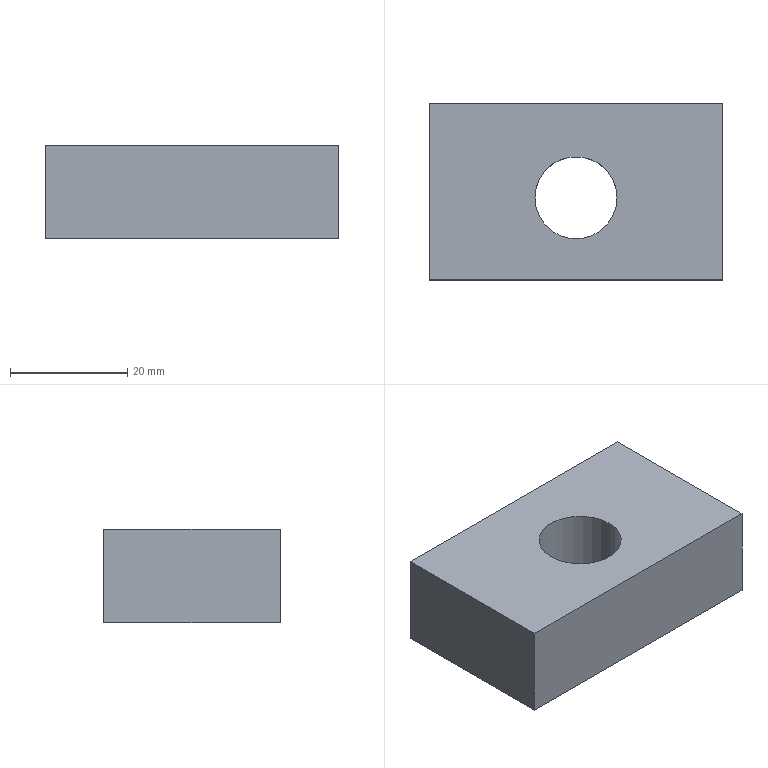Component | SolidWorks | TractionHandwheelAdjustmentPlate-1 | 1 solid | 16 faces | box 50 x 30 x 16 mm | volume 20850 mm3 | cylinder 6 | plane 6 | cone 4 | commonest cylinder face diameters 5 x4 14 x2
build123d program:
from build123d import *

# Parameters (mm, degrees)
SKETCH1_W              = 50
SKETCH1_H              = 30
EXTRUDE1_DEPTH         = 16
M6_TAPPED_HOLE1_D      = 5
M6_TAPPED_HOLE1_DEPTH  = 17
M6_TAPPED_HOLE1_TIP    = 1.502
M16_TAPPED_HOLE1_D     = 14
M16_TAPPED_HOLE1_DEPTH = 42
M16_TAPPED_HOLE1_TIP   = 4.206


with BuildPart() as part:
    # Sketch1 → Extrude1 (new body)
    with BuildSketch(Plane.XY):
        with Locations((-3.897, -9.175)):
            Rectangle(SKETCH1_W, SKETCH1_H)
    extrude(amount=EXTRUDE1_DEPTH)

    # M6 Tapped Hole1
    with Locations(Plane(origin=(0, 5.825, 0), x_dir=(-1, 0, 0), z_dir=(0, 1, 0))):
        with Locations((21.397, 8), (-13.603, 8)):
            Hole(M6_TAPPED_HOLE1_D / 2, depth=M6_TAPPED_HOLE1_DEPTH)
            with Locations((0, 0, -(M6_TAPPED_HOLE1_DEPTH + M6_TAPPED_HOLE1_TIP / 2))):  # 118° drill point
                Cone(0, M6_TAPPED_HOLE1_D / 2, M6_TAPPED_HOLE1_TIP, mode=Mode.SUBTRACT)

    # M16 Tapped Hole1
    with Locations(Plane(origin=(-3.897, -10.175, 16), x_dir=(1, 0, 0), z_dir=(0, 0, 1))):
        with Locations((0, 0)):
            Hole(M16_TAPPED_HOLE1_D / 2, depth=M16_TAPPED_HOLE1_DEPTH)
            with Locations((0, 0, -(M16_TAPPED_HOLE1_DEPTH + M16_TAPPED_HOLE1_TIP / 2))):  # 118° drill point
                Cone(0, M16_TAPPED_HOLE1_D / 2, M16_TAPPED_HOLE1_TIP, mode=Mode.SUBTRACT)


solid = part.part

# Placed as in the assembly
solid = solid.moved(Location((254.113, 482.158, -60.552), (0, 0, 0)))
STEP:
#1=CARTESIAN_POINT('',(9.575,18.582,-2.384));
#2=VERTEX_POINT('',#1);
#3=CARTESIAN_POINT('',(10.127,18.582,-2.384));
#4=VERTEX_POINT('',#3);
#5=CARTESIAN_POINT('',(9.851,18.582,-2.384));
#6=DIRECTION('',(0.,0.,1.));
#7=DIRECTION('',(1.,0.,0.));
#8=AXIS2_PLACEMENT_3D('',#5,#6,#7);
#9=CIRCLE('',#8,0.2756);
#10=EDGE_CURVE('',#2,#4,#9,.T.);
#11=ORIENTED_EDGE('',*,*,#10,.F.);
#12=CARTESIAN_POINT('',(9.575,18.582,-1.754));
#13=VERTEX_POINT('',#12);
#14=CARTESIAN_POINT('',(9.575,18.582,-1.754));
#15=DIRECTION('',(0.,0.,1.));
#16=VECTOR('',#15,39.37);
#17=LINE('',#14,#16);
#18=EDGE_CURVE('',#2,#13,#17,.T.);
#19=ORIENTED_EDGE('',*,*,#18,.T.);
#20=CARTESIAN_POINT('',(10.127,18.582,-1.754));
#21=VERTEX_POINT('',#20);
#22=CARTESIAN_POINT('',(9.851,18.582,-1.754));
#23=DIRECTION('',(0.,0.,1.));
#24=DIRECTION('',(1.,0.,0.));
#25=AXIS2_PLACEMENT_3D('',#22,#23,#24);
#26=CIRCLE('',#25,0.2756);
#27=EDGE_CURVE('',#13,#21,#26,.T.);
#28=ORIENTED_EDGE('',*,*,#27,.T.);
#29=CARTESIAN_POINT('',(10.127,18.582,-1.754));
#30=DIRECTION('',(0.,0.,1.));
#31=VECTOR('',#30,39.37);
#32=LINE('',#29,#31);
#33=EDGE_CURVE('',#4,#21,#32,.T.);
#34=ORIENTED_EDGE('',*,*,#33,.F.);
#35=EDGE_LOOP('',(#11,#19,#28,#34));
#36=FACE_OUTER_BOUND('',#35,.T.);
#37=CARTESIAN_POINT('',(9.851,18.582,-1.754));
#38=DIRECTION('',(0.,0.,1.));
#39=DIRECTION('',(1.,0.,0.));
#40=AXIS2_PLACEMENT_3D('',#37,#38,#39);
#41=CYLINDRICAL_SURFACE('',#40,0.2756);
#42=ADVANCED_FACE('',(#36),#41,.F.);
#43=CARTESIAN_POINT('',(9.162,18.543,-2.167));
#44=VERTEX_POINT('',#43);
#45=CARTESIAN_POINT('',(9.162,18.543,-1.971));
#46=VERTEX_POINT('',#45);
#47=CARTESIAN_POINT('',(9.162,18.543,-2.069));
#48=DIRECTION('',(0.,1.,0.));
#49=DIRECTION('',(0.,0.,1.));
#50=AXIS2_PLACEMENT_3D('',#47,#48,#49);
#51=CIRCLE('',#50,0.09843);
#52=EDGE_CURVE('',#44,#46,#51,.T.);
#53=ORIENTED_EDGE('',*,*,#52,.F.);
#54=CARTESIAN_POINT('',(9.162,19.212,-2.167));
#55=VERTEX_POINT('',#54);
#56=CARTESIAN_POINT('',(9.162,19.212,-2.167));
#57=DIRECTION('',(0.,1.,0.));
#58=VECTOR('',#57,39.37);
#59=LINE('',#56,#58);
#60=EDGE_CURVE('',#44,#55,#59,.T.);
#61=ORIENTED_EDGE('',*,*,#60,.T.);
#62=CARTESIAN_POINT('',(9.162,19.212,-1.971));
#63=VERTEX_POINT('',#62);
#64=CARTESIAN_POINT('',(9.162,19.212,-2.069));
#65=DIRECTION('',(0.,1.,0.));
#66=DIRECTION('',(0.,0.,1.));
#67=AXIS2_PLACEMENT_3D('',#64,#65,#66);
#68=CIRCLE('',#67,0.09843);
#69=EDGE_CURVE('',#55,#63,#68,.T.);
#70=ORIENTED_EDGE('',*,*,#69,.T.);
#71=CARTESIAN_POINT('',(9.162,19.212,-1.971));
#72=DIRECTION('',(0.,1.,0.));
#73=VECTOR('',#72,39.37);
#74=LINE('',#71,#73);
#75=EDGE_CURVE('',#46,#63,#74,.T.);
#76=ORIENTED_EDGE('',*,*,#75,.F.);
#77=EDGE_LOOP('',(#53,#61,#70,#76));
#78=FACE_OUTER_BOUND('',#77,.T.);
#79=CARTESIAN_POINT('',(9.162,19.212,-2.069));
#80=DIRECTION('',(0.,1.,0.));
#81=DIRECTION('',(0.,0.,1.));
#82=AXIS2_PLACEMENT_3D('',#79,#80,#81);
#83=CYLINDRICAL_SURFACE('',#82,0.09843);
#84=ADVANCED_FACE('',(#78),#83,.F.);
#85=CARTESIAN_POINT('',(9.162,18.484,-2.069));
#86=VERTEX_POINT('',#85);
#87=CARTESIAN_POINT('',(9.162,18.543,-1.971));
#88=DIRECTION('',(0.,0.515,0.8572));
#89=VECTOR('',#88,39.37);
#90=LINE('',#87,#89);
#91=EDGE_CURVE('',#86,#46,#90,.T.);
#92=ORIENTED_EDGE('',*,*,#91,.F.);
#93=CARTESIAN_POINT('',(9.162,18.543,-2.167));
#94=DIRECTION('',(0.,0.515,-0.8572));
#95=VECTOR('',#94,39.37);
#96=LINE('',#93,#95);
#97=EDGE_CURVE('',#86,#44,#96,.T.);
#98=ORIENTED_EDGE('',*,*,#97,.T.);
#99=ORIENTED_EDGE('',*,*,#52,.T.);
#100=EDGE_LOOP('',(#92,#98,#99));
#101=FACE_OUTER_BOUND('',#100,.T.);
#102=CARTESIAN_POINT('',(9.162,18.543,-2.069));
#103=DIRECTION('',(0.,1.,0.));
#104=DIRECTION('',(0.,0.,1.));
#105=AXIS2_PLACEMENT_3D('',#102,#103,#104);
#106=CONICAL_SURFACE('',#105,0.09843,1.03);
#107=ADVANCED_FACE('',(#101),#106,.F.);
#108=CARTESIAN_POINT('',(10.54,18.543,-2.167));
#109=VERTEX_POINT('',#108);
#110=CARTESIAN_POINT('',(10.54,18.543,-1.971));
#111=VERTEX_POINT('',#110);
#112=CARTESIAN_POINT('',(10.54,18.543,-2.069));
#113=DIRECTION('',(0.,1.,0.));
#114=DIRECTION('',(0.,0.,1.));
#115=AXIS2_PLACEMENT_3D('',#112,#113,#114);
#116=CIRCLE('',#115,0.09843);
#117=EDGE_CURVE('',#109,#111,#116,.T.);
#118=ORIENTED_EDGE('',*,*,#117,.F.);
#119=CARTESIAN_POINT('',(10.54,19.212,-2.167));
#120=VERTEX_POINT('',#119);
#121=CARTESIAN_POINT('',(10.54,19.212,-2.167));
#122=DIRECTION('',(0.,1.,0.));
#123=VECTOR('',#122,39.37);
#124=LINE('',#121,#123);
#125=EDGE_CURVE('',#109,#120,#124,.T.);
#126=ORIENTED_EDGE('',*,*,#125,.T.);
#127=CARTESIAN_POINT('',(10.54,19.212,-1.971));
#128=VERTEX_POINT('',#127);
#129=CARTESIAN_POINT('',(10.54,19.212,-2.069));
#130=DIRECTION('',(0.,1.,0.));
#131=DIRECTION('',(0.,0.,1.));
#132=AXIS2_PLACEMENT_3D('',#129,#130,#131);
#133=CIRCLE('',#132,0.09843);
#134=EDGE_CURVE('',#120,#128,#133,.T.);
#135=ORIENTED_EDGE('',*,*,#134,.T.);
#136=CARTESIAN_POINT('',(10.54,19.212,-1.971));
#137=DIRECTION('',(0.,1.,0.));
#138=VECTOR('',#137,39.37);
#139=LINE('',#136,#138);
#140=EDGE_CURVE('',#111,#128,#139,.T.);
#141=ORIENTED_EDGE('',*,*,#140,.F.);
#142=EDGE_LOOP('',(#118,#126,#135,#141));
#143=FACE_OUTER_BOUND('',#142,.T.);
#144=CARTESIAN_POINT('',(10.54,19.212,-2.069));
#145=DIRECTION('',(0.,1.,0.));
#146=DIRECTION('',(0.,0.,1.));
#147=AXIS2_PLACEMENT_3D('',#144,#145,#146);
#148=CYLINDRICAL_SURFACE('',#147,0.09843);
#149=ADVANCED_FACE('',(#143),#148,.F.);
#150=CARTESIAN_POINT('',(10.54,18.484,-2.069));
#151=VERTEX_POINT('',#150);
#152=CARTESIAN_POINT('',(10.54,18.543,-1.971));
#153=DIRECTION('',(0.,0.515,0.8572));
#154=VECTOR('',#153,39.37);
#155=LINE('',#152,#154);
#156=EDGE_CURVE('',#151,#111,#155,.T.);
#157=ORIENTED_EDGE('',*,*,#156,.F.);
#158=CARTESIAN_POINT('',(10.54,18.543,-2.167));
#159=DIRECTION('',(0.,0.515,-0.8572));
#160=VECTOR('',#159,39.37);
#161=LINE('',#158,#160);
#162=EDGE_CURVE('',#151,#109,#161,.T.);
#163=ORIENTED_EDGE('',*,*,#162,.T.);
#164=ORIENTED_EDGE('',*,*,#117,.T.);
#165=EDGE_LOOP('',(#157,#163,#164));
#166=FACE_OUTER_BOUND('',#165,.T.);
#167=CARTESIAN_POINT('',(10.54,18.543,-2.069));
#168=DIRECTION('',(0.,1.,0.));
#169=DIRECTION('',(0.,0.,1.));
#170=AXIS2_PLACEMENT_3D('',#167,#168,#169);
#171=CONICAL_SURFACE('',#170,0.09843,1.03);
#172=ADVANCED_FACE('',(#166),#171,.F.);
#173=CARTESIAN_POINT('',(8.867,19.212,-2.384));
#174=VERTEX_POINT('',#173);
#175=CARTESIAN_POINT('',(8.867,18.031,-2.384));
#176=VERTEX_POINT('',#175);
#177=CARTESIAN_POINT('',(8.867,19.212,-2.384));
#178=DIRECTION('',(0.,-1.,0.));
#179=VECTOR('',#178,39.37);
#180=LINE('',#177,#179);
#181=EDGE_CURVE('',#174,#176,#180,.T.);
#182=ORIENTED_EDGE('',*,*,#181,.T.);
#183=CARTESIAN_POINT('',(8.867,18.031,-1.754));
#184=VERTEX_POINT('',#183);
#185=CARTESIAN_POINT('',(8.867,18.031,-1.754));
#186=DIRECTION('',(0.,0.,-1.));
#187=VECTOR('',#186,39.37);
#188=LINE('',#185,#187);
#189=EDGE_CURVE('',#184,#176,#188,.T.);
#190=ORIENTED_EDGE('',*,*,#189,.F.);
#191=CARTESIAN_POINT('',(8.867,19.212,-1.754));
#192=VERTEX_POINT('',#191);
#193=CARTESIAN_POINT('',(8.867,19.212,-1.754));
#194=DIRECTION('',(0.,-1.,0.));
#195=VECTOR('',#194,39.37);
#196=LINE('',#193,#195);
#197=EDGE_CURVE('',#192,#184,#196,.T.);
#198=ORIENTED_EDGE('',*,*,#197,.F.);
#199=CARTESIAN_POINT('',(8.867,19.212,-1.754));
#200=DIRECTION('',(0.,0.,-1.));
#201=VECTOR('',#200,39.37);
#202=LINE('',#199,#201);
#203=EDGE_CURVE('',#192,#174,#202,.T.);
#204=ORIENTED_EDGE('',*,*,#203,.T.);
#205=EDGE_LOOP('',(#182,#190,#198,#204));
#206=FACE_OUTER_BOUND('',#205,.T.);
#207=CARTESIAN_POINT('',(8.867,19.212,-1.754));
#208=DIRECTION('',(1.,0.,0.));
#209=DIRECTION('',(-0.,1.,0.));
#210=AXIS2_PLACEMENT_3D('',#207,#208,#209);
#211=PLANE('',#210);
#212=ADVANCED_FACE('',(#206),#211,.F.);
#213=CARTESIAN_POINT('',(10.835,18.031,-2.384));
#214=VERTEX_POINT('',#213);
#215=CARTESIAN_POINT('',(8.867,18.031,-2.384));
#216=DIRECTION('',(1.,0.,0.));
#217=VECTOR('',#216,39.37);
#218=LINE('',#215,#217);
#219=EDGE_CURVE('',#176,#214,#218,.T.);
#220=ORIENTED_EDGE('',*,*,#219,.T.);
#221=CARTESIAN_POINT('',(10.835,18.031,-1.754));
#222=VERTEX_POINT('',#221);
#223=CARTESIAN_POINT('',(10.835,18.031,-1.754));
#224=DIRECTION('',(0.,0.,-1.));
#225=VECTOR('',#224,39.37);
#226=LINE('',#223,#225);
#227=EDGE_CURVE('',#222,#214,#226,.T.);
#228=ORIENTED_EDGE('',*,*,#227,.F.);
#229=CARTESIAN_POINT('',(8.867,18.031,-1.754));
#230=DIRECTION('',(1.,0.,0.));
#231=VECTOR('',#230,39.37);
#232=LINE('',#229,#231);
#233=EDGE_CURVE('',#184,#222,#232,.T.);
#234=ORIENTED_EDGE('',*,*,#233,.F.);
#235=ORIENTED_EDGE('',*,*,#189,.T.);
#236=EDGE_LOOP('',(#220,#228,#234,#235));
#237=FACE_OUTER_BOUND('',#236,.T.);
#238=CARTESIAN_POINT('',(8.867,18.031,-1.754));
#239=DIRECTION('',(0.,1.,0.));
#240=DIRECTION('',(0.,0.,1.));
#241=AXIS2_PLACEMENT_3D('',#238,#239,#240);
#242=PLANE('',#241);
#243=ADVANCED_FACE('',(#237),#242,.F.);
#244=CARTESIAN_POINT('',(10.835,19.212,-2.384));
#245=VERTEX_POINT('',#244);
#246=CARTESIAN_POINT('',(10.835,19.212,-2.384));
#247=DIRECTION('',(-0.,1.,0.));
#248=VECTOR('',#247,39.37);
#249=LINE('',#246,#248);
#250=EDGE_CURVE('',#214,#245,#249,.T.);
#251=ORIENTED_EDGE('',*,*,#250,.T.);
#252=CARTESIAN_POINT('',(10.835,19.212,-1.754));
#253=VERTEX_POINT('',#252);
#254=CARTESIAN_POINT('',(10.835,19.212,-1.754));
#255=DIRECTION('',(0.,0.,-1.));
#256=VECTOR('',#255,39.37);
#257=LINE('',#254,#256);
#258=EDGE_CURVE('',#253,#245,#257,.T.);
#259=ORIENTED_EDGE('',*,*,#258,.F.);
#260=CARTESIAN_POINT('',(10.835,19.212,-1.754));
#261=DIRECTION('',(-0.,1.,0.));
#262=VECTOR('',#261,39.37);
#263=LINE('',#260,#262);
#264=EDGE_CURVE('',#222,#253,#263,.T.);
#265=ORIENTED_EDGE('',*,*,#264,.F.);
#266=ORIENTED_EDGE('',*,*,#227,.T.);
#267=EDGE_LOOP('',(#251,#259,#265,#266));
#268=FACE_OUTER_BOUND('',#267,.T.);
#269=CARTESIAN_POINT('',(10.835,19.212,-1.754));
#270=DIRECTION('',(-1.,-0.,0.));
#271=DIRECTION('',(0.,-1.,0.));
#272=AXIS2_PLACEMENT_3D('',#269,#270,#271);
#273=PLANE('',#272);
#274=ADVANCED_FACE('',(#268),#273,.F.);
#275=CARTESIAN_POINT('',(9.162,19.212,-2.069));
#276=DIRECTION('',(0.,1.,0.));
#277=DIRECTION('',(0.,0.,1.));
#278=AXIS2_PLACEMENT_3D('',#275,#276,#277);
#279=CIRCLE('',#278,0.09843);
#280=EDGE_CURVE('',#63,#55,#279,.T.);
#281=ORIENTED_EDGE('',*,*,#280,.F.);
#282=ORIENTED_EDGE('',*,*,#69,.F.);
#283=EDGE_LOOP('',(#281,#282));
#284=FACE_BOUND('',#283,.T.);
#285=CARTESIAN_POINT('',(10.54,19.212,-2.069));
#286=DIRECTION('',(0.,1.,0.));
#287=DIRECTION('',(0.,0.,1.));
#288=AXIS2_PLACEMENT_3D('',#285,#286,#287);
#289=CIRCLE('',#288,0.09843);
#290=EDGE_CURVE('',#128,#120,#289,.T.);
#291=ORIENTED_EDGE('',*,*,#290,.F.);
#292=ORIENTED_EDGE('',*,*,#134,.F.);
#293=EDGE_LOOP('',(#291,#292));
#294=FACE_BOUND('',#293,.T.);
#295=CARTESIAN_POINT('',(8.867,19.212,-2.384));
#296=DIRECTION('',(-1.,0.,0.));
#297=VECTOR('',#296,39.37);
#298=LINE('',#295,#297);
#299=EDGE_CURVE('',#245,#174,#298,.T.);
#300=ORIENTED_EDGE('',*,*,#299,.T.);
#301=ORIENTED_EDGE('',*,*,#203,.F.);
#302=CARTESIAN_POINT('',(8.867,19.212,-1.754));
#303=DIRECTION('',(-1.,0.,0.));
#304=VECTOR('',#303,39.37);
#305=LINE('',#302,#304);
#306=EDGE_CURVE('',#253,#192,#305,.T.);
#307=ORIENTED_EDGE('',*,*,#306,.F.);
#308=ORIENTED_EDGE('',*,*,#258,.T.);
#309=EDGE_LOOP('',(#300,#301,#307,#308));
#310=FACE_OUTER_BOUND('',#309,.T.);
#311=CARTESIAN_POINT('',(8.867,19.212,-1.754));
#312=DIRECTION('',(0.,-1.,0.));
#313=DIRECTION('',(0.,0.,-1.));
#314=AXIS2_PLACEMENT_3D('',#311,#312,#313);
#315=PLANE('',#314);
#316=ADVANCED_FACE('',(#284,#294,#310),#315,.F.);
#317=CARTESIAN_POINT('',(9.851,18.582,-1.754));
#318=DIRECTION('',(0.,0.,1.));
#319=DIRECTION('',(1.,0.,0.));
#320=AXIS2_PLACEMENT_3D('',#317,#318,#319);
#321=CIRCLE('',#320,0.2756);
#322=EDGE_CURVE('',#21,#13,#321,.T.);
#323=ORIENTED_EDGE('',*,*,#322,.F.);
#324=ORIENTED_EDGE('',*,*,#27,.F.);
#325=EDGE_LOOP('',(#323,#324));
#326=FACE_BOUND('',#325,.T.);
#327=ORIENTED_EDGE('',*,*,#197,.T.);
#328=ORIENTED_EDGE('',*,*,#233,.T.);
#329=ORIENTED_EDGE('',*,*,#264,.T.);
#330=ORIENTED_EDGE('',*,*,#306,.T.);
#331=EDGE_LOOP('',(#327,#328,#329,#330));
#332=FACE_OUTER_BOUND('',#331,.T.);
#333=CARTESIAN_POINT('',(8.867,18.031,-1.754));
#334=DIRECTION('',(0.,0.,1.));
#335=DIRECTION('',(1.,0.,0.));
#336=AXIS2_PLACEMENT_3D('',#333,#334,#335);
#337=PLANE('',#336);
#338=ADVANCED_FACE('',(#326,#332),#337,.T.);
#339=CARTESIAN_POINT('',(9.851,18.582,-2.384));
#340=DIRECTION('',(0.,0.,1.));
#341=DIRECTION('',(1.,0.,0.));
#342=AXIS2_PLACEMENT_3D('',#339,#340,#341);
#343=CIRCLE('',#342,0.2756);
#344=EDGE_CURVE('',#4,#2,#343,.T.);
#345=ORIENTED_EDGE('',*,*,#344,.T.);
#346=ORIENTED_EDGE('',*,*,#10,.T.);
#347=EDGE_LOOP('',(#345,#346));
#348=FACE_BOUND('',#347,.T.);
#349=ORIENTED_EDGE('',*,*,#181,.F.);
#350=ORIENTED_EDGE('',*,*,#299,.F.);
#351=ORIENTED_EDGE('',*,*,#250,.F.);
#352=ORIENTED_EDGE('',*,*,#219,.F.);
#353=EDGE_LOOP('',(#349,#350,#351,#352));
#354=FACE_OUTER_BOUND('',#353,.T.);
#355=CARTESIAN_POINT('',(8.867,18.031,-2.384));
#356=DIRECTION('',(0.,0.,1.));
#357=DIRECTION('',(1.,0.,0.));
#358=AXIS2_PLACEMENT_3D('',#355,#356,#357);
#359=PLANE('',#358);
#360=ADVANCED_FACE('',(#348,#354),#359,.F.);
#361=ORIENTED_EDGE('',*,*,#162,.F.);
#362=ORIENTED_EDGE('',*,*,#156,.T.);
#363=CARTESIAN_POINT('',(10.54,18.543,-2.069));
#364=DIRECTION('',(0.,1.,0.));
#365=DIRECTION('',(0.,0.,1.));
#366=AXIS2_PLACEMENT_3D('',#363,#364,#365);
#367=CIRCLE('',#366,0.09843);
#368=EDGE_CURVE('',#111,#109,#367,.T.);
#369=ORIENTED_EDGE('',*,*,#368,.T.);
#370=EDGE_LOOP('',(#361,#362,#369));
#371=FACE_OUTER_BOUND('',#370,.T.);
#372=CARTESIAN_POINT('',(10.54,18.543,-2.069));
#373=DIRECTION('',(0.,1.,0.));
#374=DIRECTION('',(0.,0.,1.));
#375=AXIS2_PLACEMENT_3D('',#372,#373,#374);
#376=CONICAL_SURFACE('',#375,0.09843,1.03);
#377=ADVANCED_FACE('',(#371),#376,.F.);
#378=ORIENTED_EDGE('',*,*,#125,.F.);
#379=ORIENTED_EDGE('',*,*,#368,.F.);
#380=ORIENTED_EDGE('',*,*,#140,.T.);
#381=ORIENTED_EDGE('',*,*,#290,.T.);
#382=EDGE_LOOP('',(#378,#379,#380,#381));
#383=FACE_OUTER_BOUND('',#382,.T.);
#384=CARTESIAN_POINT('',(10.54,19.212,-2.069));
#385=DIRECTION('',(0.,1.,0.));
#386=DIRECTION('',(0.,0.,1.));
#387=AXIS2_PLACEMENT_3D('',#384,#385,#386);
#388=CYLINDRICAL_SURFACE('',#387,0.09843);
#389=ADVANCED_FACE('',(#383),#388,.F.);
#390=ORIENTED_EDGE('',*,*,#97,.F.);
#391=ORIENTED_EDGE('',*,*,#91,.T.);
#392=CARTESIAN_POINT('',(9.162,18.543,-2.069));
#393=DIRECTION('',(0.,1.,0.));
#394=DIRECTION('',(0.,0.,1.));
#395=AXIS2_PLACEMENT_3D('',#392,#393,#394);
#396=CIRCLE('',#395,0.09843);
#397=EDGE_CURVE('',#46,#44,#396,.T.);
#398=ORIENTED_EDGE('',*,*,#397,.T.);
#399=EDGE_LOOP('',(#390,#391,#398));
#400=FACE_OUTER_BOUND('',#399,.T.);
#401=CARTESIAN_POINT('',(9.162,18.543,-2.069));
#402=DIRECTION('',(0.,1.,0.));
#403=DIRECTION('',(0.,0.,1.));
#404=AXIS2_PLACEMENT_3D('',#401,#402,#403);
#405=CONICAL_SURFACE('',#404,0.09843,1.03);
#406=ADVANCED_FACE('',(#400),#405,.F.);
#407=ORIENTED_EDGE('',*,*,#60,.F.);
#408=ORIENTED_EDGE('',*,*,#397,.F.);
#409=ORIENTED_EDGE('',*,*,#75,.T.);
#410=ORIENTED_EDGE('',*,*,#280,.T.);
#411=EDGE_LOOP('',(#407,#408,#409,#410));
#412=FACE_OUTER_BOUND('',#411,.T.);
#413=CARTESIAN_POINT('',(9.162,19.212,-2.069));
#414=DIRECTION('',(0.,1.,0.));
#415=DIRECTION('',(0.,0.,1.));
#416=AXIS2_PLACEMENT_3D('',#413,#414,#415);
#417=CYLINDRICAL_SURFACE('',#416,0.09843);
#418=ADVANCED_FACE('',(#412),#417,.F.);
#419=ORIENTED_EDGE('',*,*,#18,.F.);
#420=ORIENTED_EDGE('',*,*,#344,.F.);
#421=ORIENTED_EDGE('',*,*,#33,.T.);
#422=ORIENTED_EDGE('',*,*,#322,.T.);
#423=EDGE_LOOP('',(#419,#420,#421,#422));
#424=FACE_OUTER_BOUND('',#423,.T.);
#425=CARTESIAN_POINT('',(9.851,18.582,-1.754));
#426=DIRECTION('',(0.,0.,1.));
#427=DIRECTION('',(1.,0.,0.));
#428=AXIS2_PLACEMENT_3D('',#425,#426,#427);
#429=CYLINDRICAL_SURFACE('',#428,0.2756);
#430=ADVANCED_FACE('',(#424),#429,.F.);
#431=CLOSED_SHELL('',(#42,#84,#107,#149,#172,#212,#243,#274,#316,#338,#360,#377,#389,#406,#418,#430));
#432=MANIFOLD_SOLID_BREP('',#431);
#433=CARTESIAN_POINT('',(0.,0.,0.));
#434=DIRECTION('',(0.,0.,1.));
#435=DIRECTION('',(1.,0.,0.));
#436=AXIS2_PLACEMENT_3D('',#433,#434,#435);
#437=(LENGTH_UNIT()NAMED_UNIT(*)SI_UNIT($,.METRE.));
#438=LENGTH_MEASURE_WITH_UNIT(LENGTH_MEASURE(0.0254),#437);
#439=DIMENSIONAL_EXPONENTS(1.,0.,0.,0.,0.,0.,0.);
#440=(CONVERSION_BASED_UNIT('',#438)LENGTH_UNIT()NAMED_UNIT(#439));
#441=UNCERTAINTY_MEASURE_WITH_UNIT(LENGTH_MEASURE(0.00001),#440,'','');
#442=(NAMED_UNIT(*)PLANE_ANGLE_UNIT()SI_UNIT($,.RADIAN.));
#443=(NAMED_UNIT(*)SI_UNIT($,.STERADIAN.)SOLID_ANGLE_UNIT());
#444=(GEOMETRIC_REPRESENTATION_CONTEXT(3)GLOBAL_UNCERTAINTY_ASSIGNED_CONTEXT((#441))GLOBAL_UNIT_ASSIGNED_CONTEXT((#440,#442,#443))REPRESENTATION_CONTEXT('',''));
#445=ADVANCED_BREP_SHAPE_REPRESENTATION('',(#432,#436),#444);
#446=COLOUR_RGB('',0.7922,0.8196,0.9333);
#447=FILL_AREA_STYLE_COLOUR('',#446);
#448=FILL_AREA_STYLE('',(#447));
#449=SURFACE_STYLE_FILL_AREA(#448);
#450=SURFACE_SIDE_STYLE('',(#449));
#451=SURFACE_STYLE_USAGE(.BOTH.,#450);
#452=PRESENTATION_STYLE_ASSIGNMENT((#451));
#453=STYLED_ITEM('',(#452),#432);
#454=(LENGTH_UNIT()NAMED_UNIT(*)SI_UNIT($,.METRE.));
#455=LENGTH_MEASURE_WITH_UNIT(LENGTH_MEASURE(0.0254),#454);
#456=DIMENSIONAL_EXPONENTS(1.,0.,0.,0.,0.,0.,0.);
#457=(CONVERSION_BASED_UNIT('',#455)LENGTH_UNIT()NAMED_UNIT(#456));
#458=UNCERTAINTY_MEASURE_WITH_UNIT(LENGTH_MEASURE(0.00001),#457,'','');
#459=(NAMED_UNIT(*)PLANE_ANGLE_UNIT()SI_UNIT($,.RADIAN.));
#460=(NAMED_UNIT(*)SI_UNIT($,.STERADIAN.)SOLID_ANGLE_UNIT());
#461=(GEOMETRIC_REPRESENTATION_CONTEXT(3)GLOBAL_UNCERTAINTY_ASSIGNED_CONTEXT((#458))GLOBAL_UNIT_ASSIGNED_CONTEXT((#457,#459,#460))REPRESENTATION_CONTEXT('',''));
#462=MECHANICAL_DESIGN_GEOMETRIC_PRESENTATION_REPRESENTATION('',(#453),#461);
#463=PRESENTATION_LAYER_ASSIGNMENT('','',(#453));